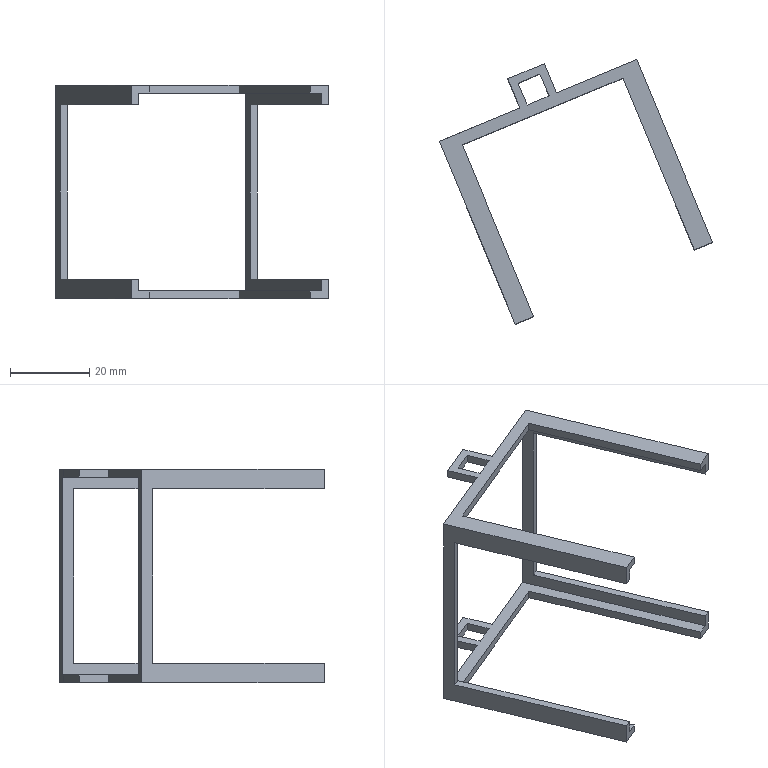Component | SolidWorks | BatteryExoskeleton-1 | 1 solid | 40 faces | box 69.03 x 66.87 x 54 mm | volume 4432 mm3 | plane 40
build123d program:
from build123d import *

# Parameters (mm, degrees)
SKETCH1_W           = 54
SKETCH1_H           = 54
SKETCH1_W_2         = 50
SKETCH1_H_2         = 50
BOSS_EXTRUDE1_DEPTH = 50
CUT_EXTRUDE2_REACH  = 80.875
SKETCH3_W           = 44
SKETCH3_H           = 144
CUT_EXTRUDE3_DEPTH  = 150
CUT_EXTRUDE4_DEPTH  = 150
BOSS_EXTRUDE3_DEPTH = 2
BOSS_EXTRUDE4_DEPTH = 2


with BuildPart() as part:
    # Sketch1 → Boss-Extrude1 (new body)
    with BuildSketch(Plane.XY):
        with Locations((1.279, -1.377)):
            Rectangle(SKETCH1_W, SKETCH1_H)
        with Locations((1.279, -1.377)):
            Rectangle(SKETCH1_W_2, SKETCH1_H_2, mode=Mode.SUBTRACT)
    extrude(amount=BOSS_EXTRUDE1_DEPTH)

    # Sketch2 → Cut-Extrude2 (cut, up to next)
    with BuildSketch(Plane.ZY.offset(25.721), mode=Mode.PRIVATE) as cut_extrude2_sk1:
        Polygon((145, -23.377), (5, -23.377), (3, -23.377), (3, 20.623), (5, 20.623), (145, 20.623), (147, 20.623), (147, -23.377), align=None)
    cut_extrude2_tool1 = extrude(cut_extrude2_sk1.sketch, amount=-CUT_EXTRUDE2_REACH, mode=Mode.PRIVATE) & part.part
    add(cut_extrude2_tool1.solids().sort_by_distance((-25.721, -1.377, 75))[0], mode=Mode.SUBTRACT)

    # Sketch3 → Cut-Extrude3 (cut)
    with BuildSketch(Plane(origin=(0, 25.623, 0), x_dir=(1, 0, 0), z_dir=(0, 1, 0))):
        with Locations((1.279, -75)):
            Rectangle(SKETCH3_W, SKETCH3_H)
    extrude(amount=-CUT_EXTRUDE3_DEPTH, mode=Mode.SUBTRACT)

    # Sketch4 → Cut-Extrude4 (cut)
    with BuildSketch(Plane(origin=(28.279, 0, 0), x_dir=(0, 0, -1), z_dir=(1, 0, 0))):
        Polygon((-147, 20.623), (-147, -23.377), (-145, -23.377), (-5, -23.377), (-3, -23.377), (-3, 20.623), (-5, 20.623), (-145, 20.623), align=None)
    extrude(amount=-CUT_EXTRUDE4_DEPTH, mode=Mode.SUBTRACT)

    # Sketch7 → Boss-Extrude3 (add)
    with BuildSketch(Plane.XZ.offset(28.377)):
        Polygon((-3.72, 0), (-3.72, -8), (6.28, -8), (6.28, 0), (4.28, 0), (4.28, -6), (-1.72, -6), (-1.72, 0), align=None)
    extrude(amount=-BOSS_EXTRUDE3_DEPTH)

    # Sketch8 → Boss-Extrude4 (add)
    with BuildSketch(Plane(origin=(0, 25.623, 0), x_dir=(1, 0, 0), z_dir=(0, 1, 0))):
        Polygon((-3.72, 0), (-1.72, 0), (-1.72, 6), (4.28, 6), (4.28, 0), (6.28, 0), (6.28, 8), (-3.72, 8), align=None)
    extrude(amount=-BOSS_EXTRUDE4_DEPTH)


solid = part.part

# Placed as in the assembly
solid = solid.moved(Location((22.48, 30.643, 269.469), (90, 22.523, 180)))